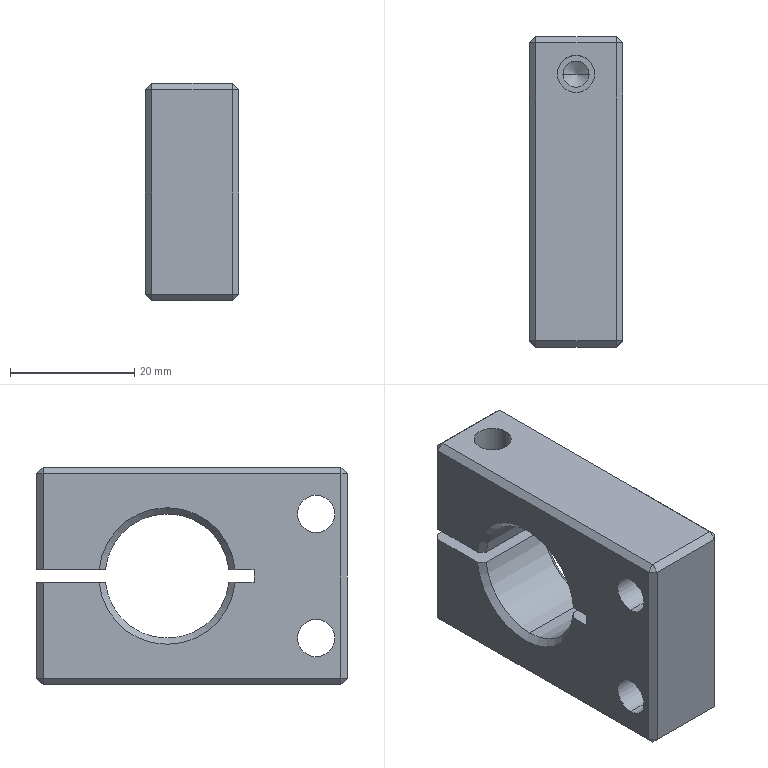Component | SolidWorks | TC020.05-01-1 | 1 solid | 53 faces | volume 19318 mm3 | plane 34 | cylinder 11 | cone 8 | commonest cylinder face diameters 6 x6 20 x3 4.2 x2 | material Q235A